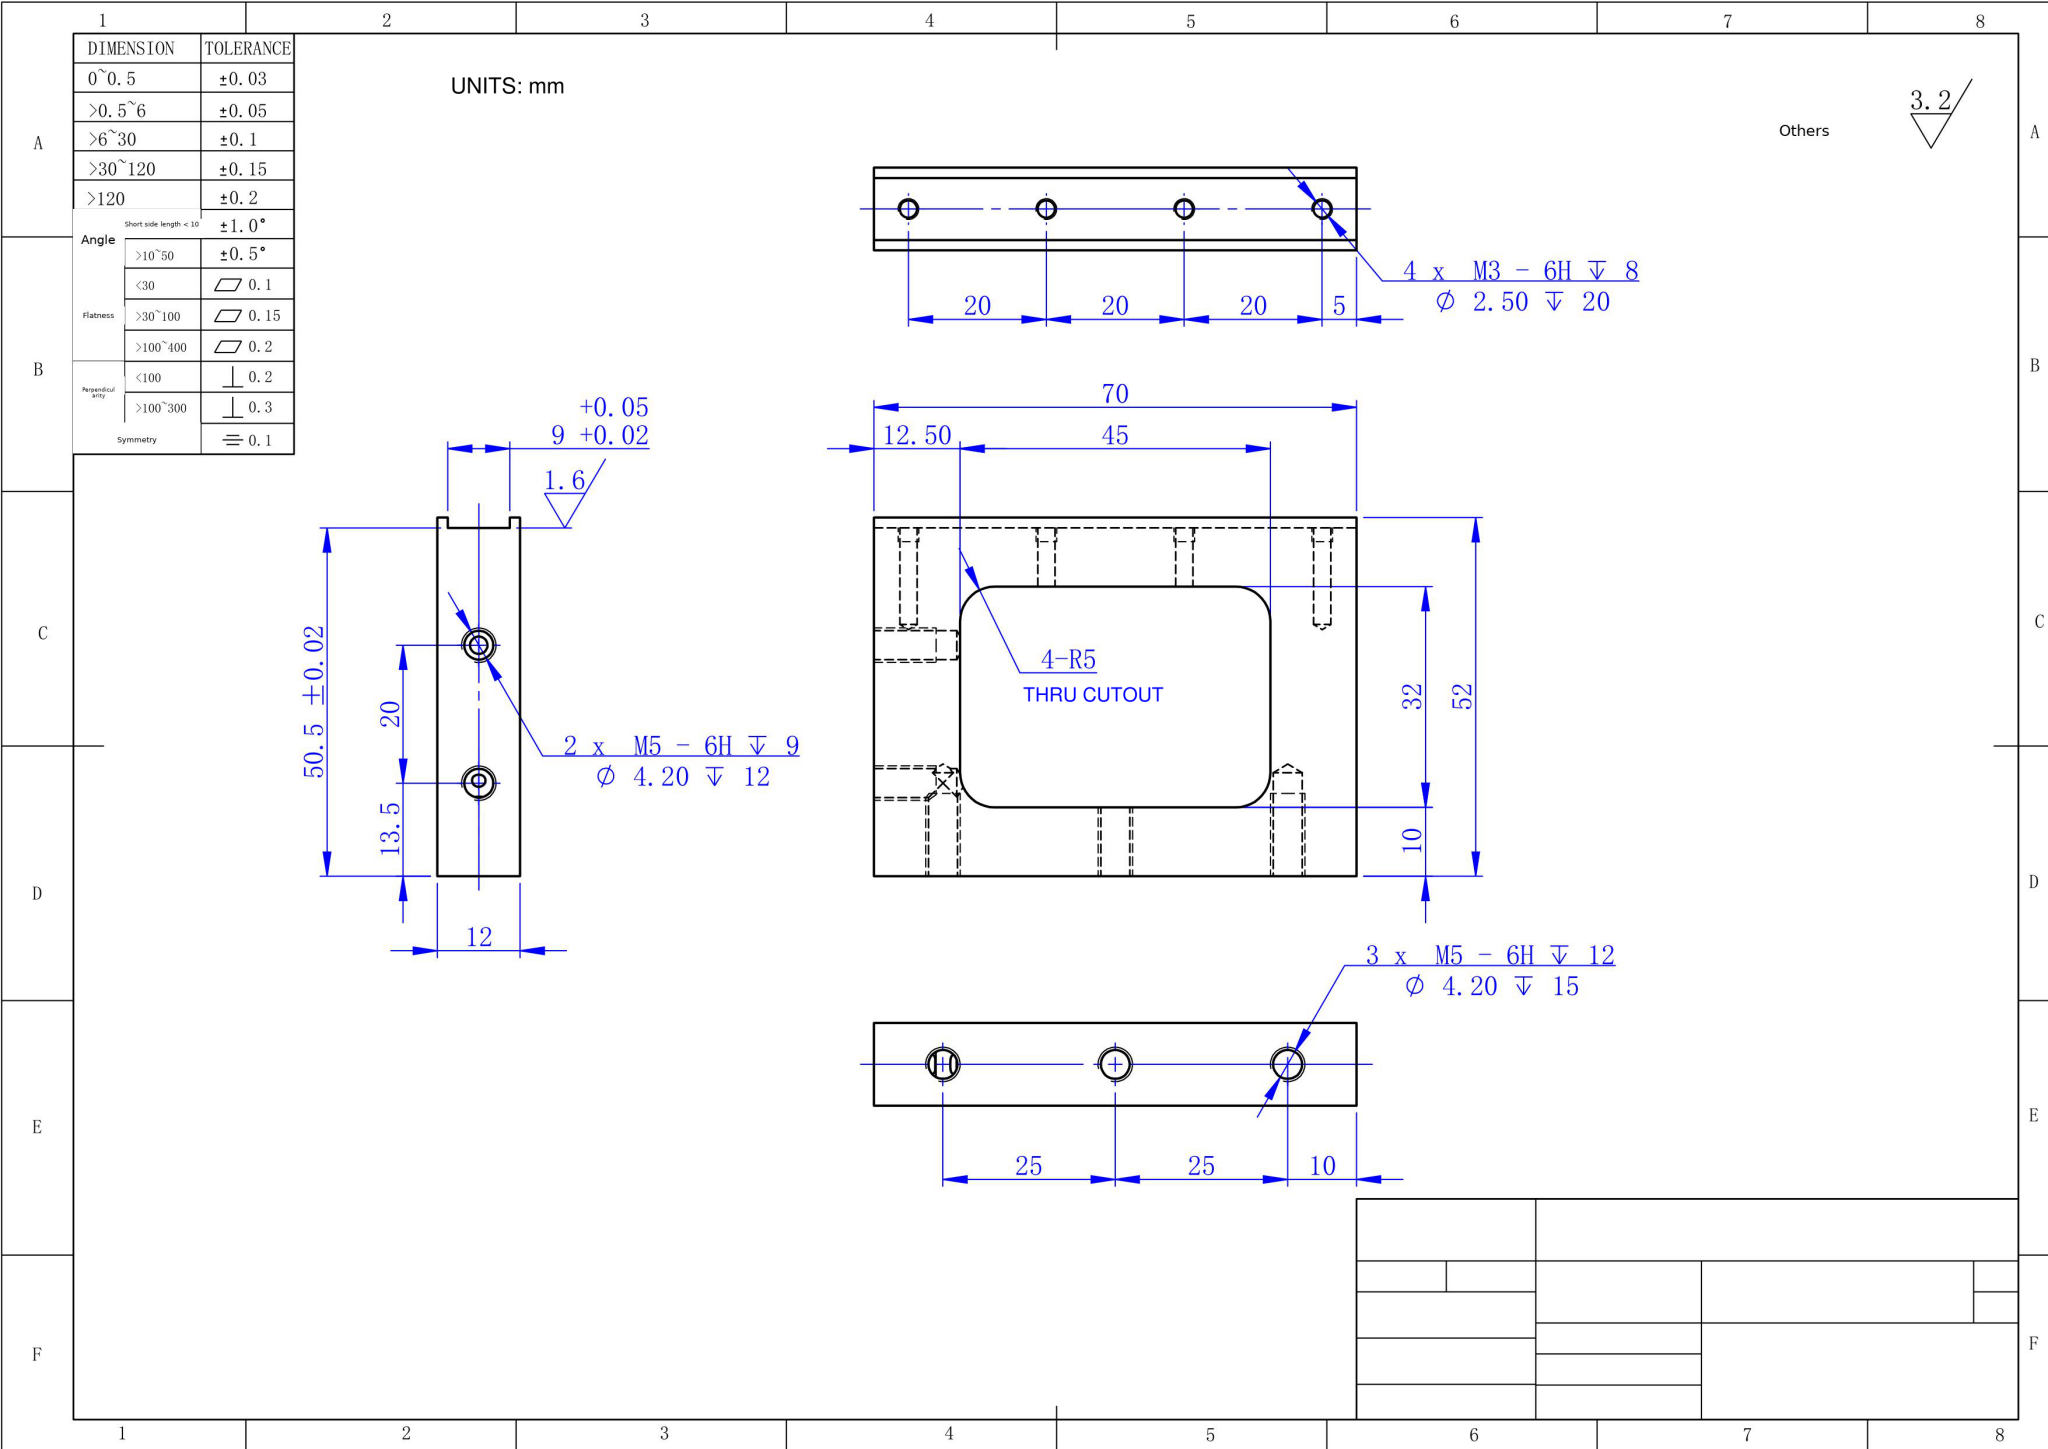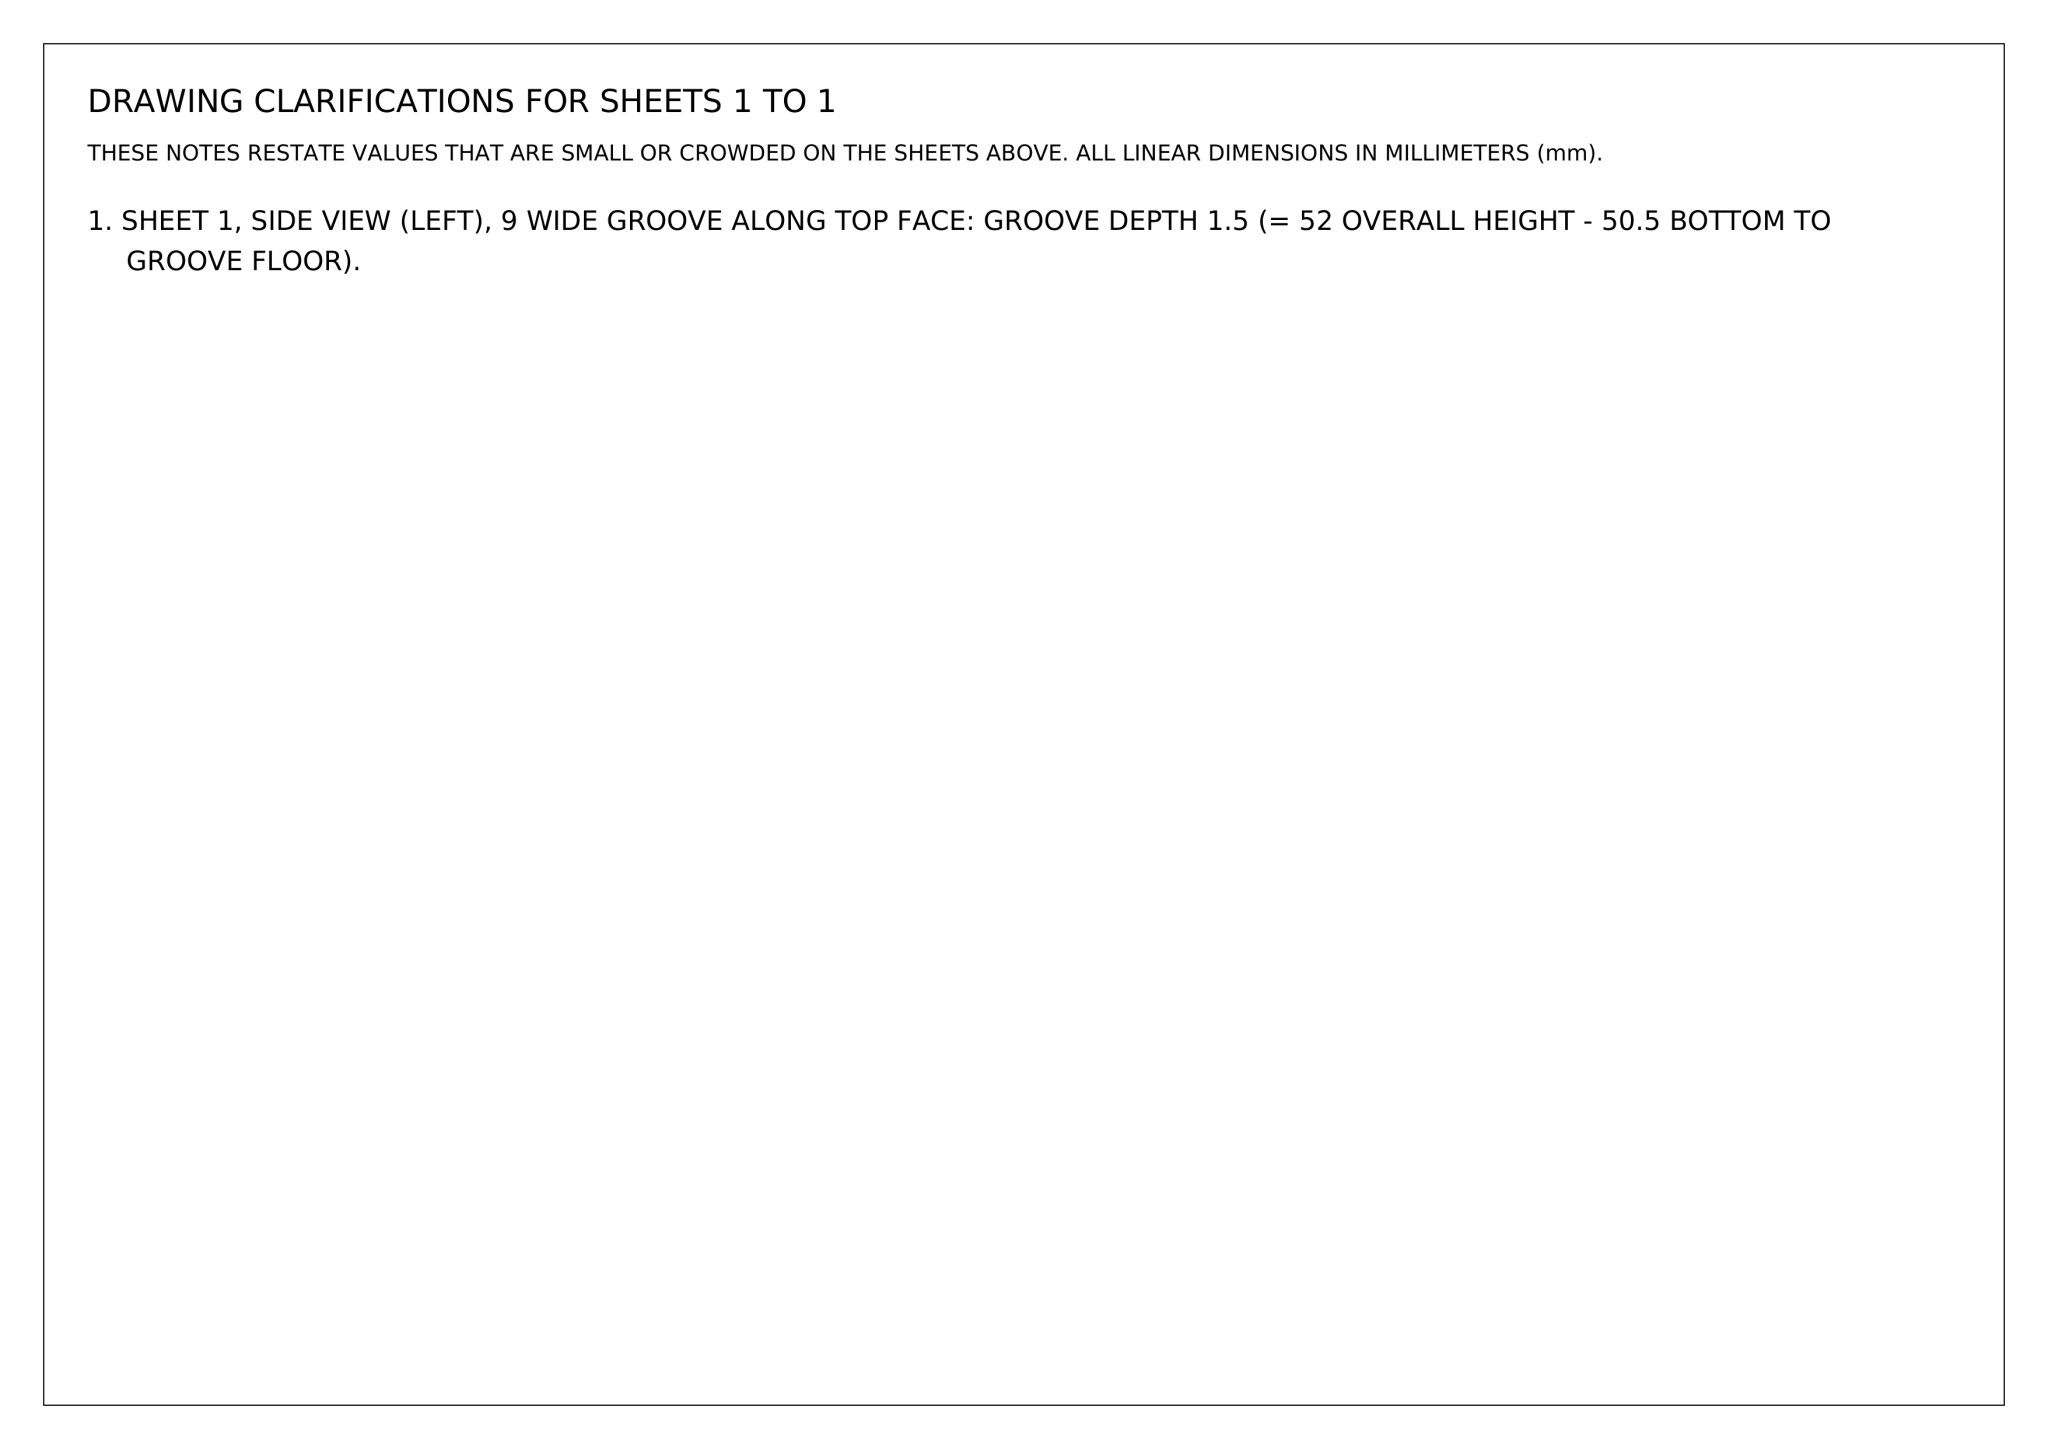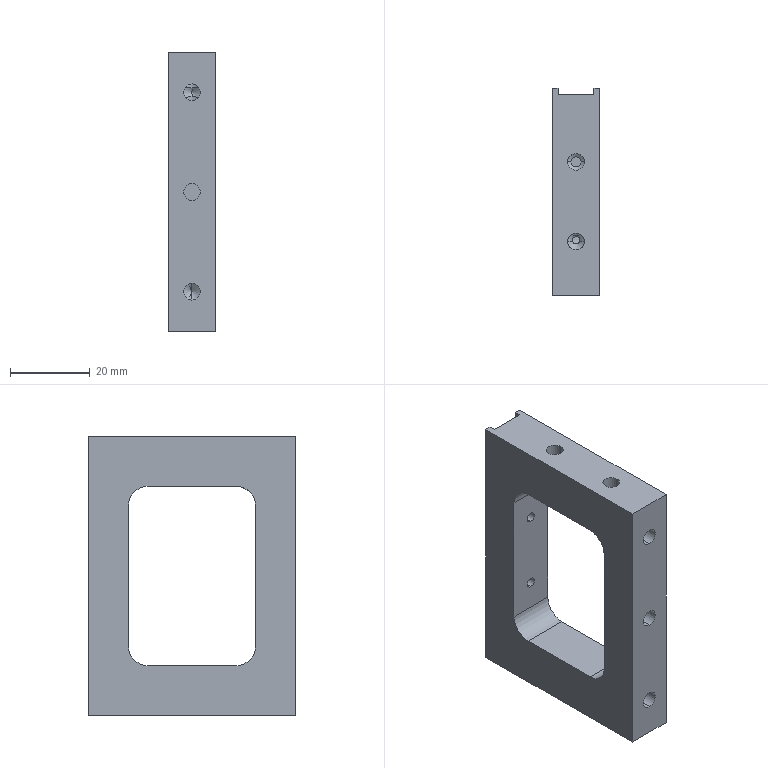Part | NX | mm | 1 solid | 53 faces | box 12 x 52 x 70 mm | volume 24629 mm3 | cylinder 27 | plane 14 | cone 12 | commonest cylinder face diameters 4.2 x15 2.5 x8 10 x4